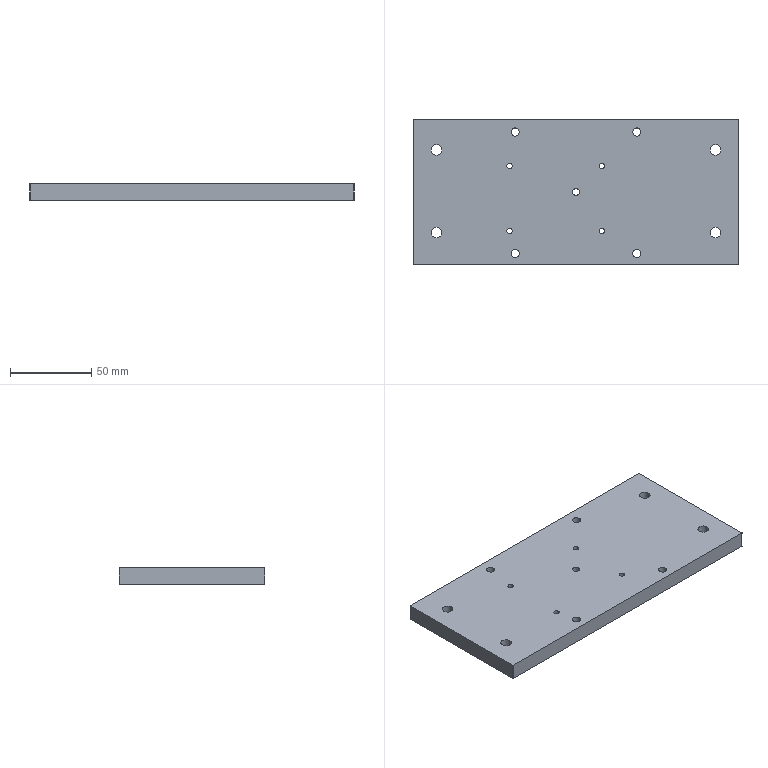CAM job | Mastercam | mm | 8 operations | part box 200 x 90 x 10
1. Facing | 20 - 63 平铣刀
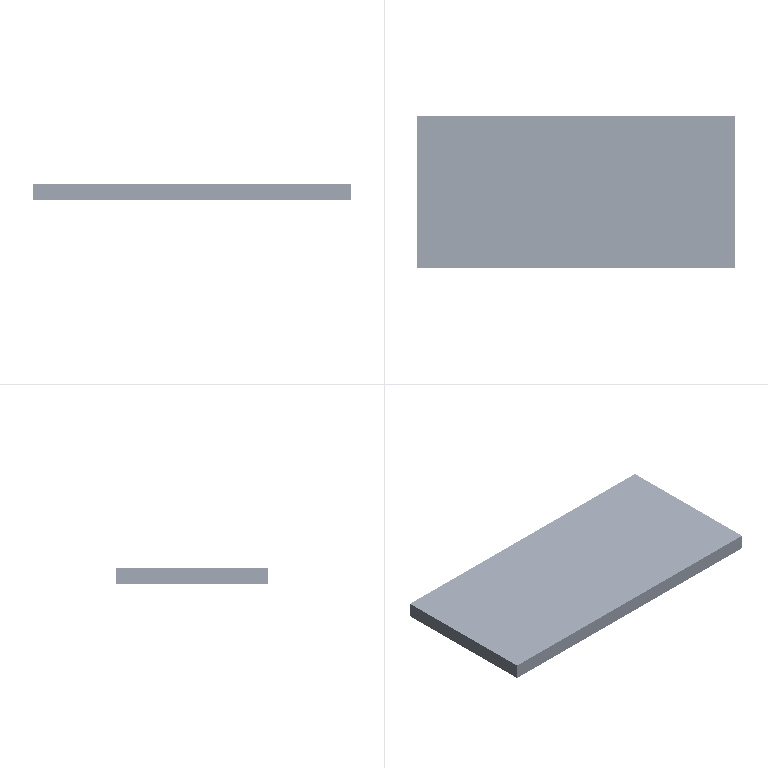2. Contour (Ramp) | 12 - 12 平铣刀
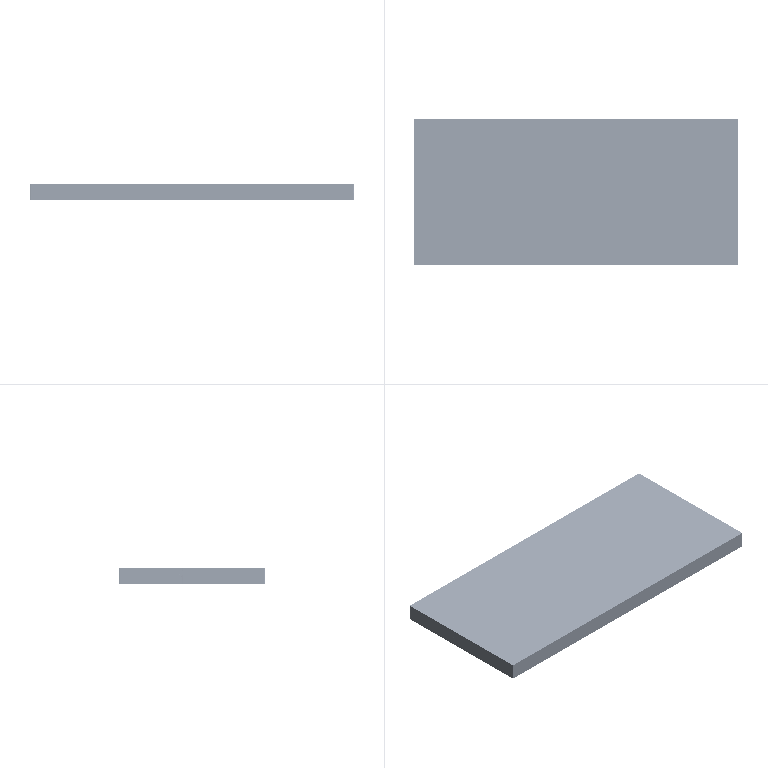3. Contour (2D) | 12 - 12 平铣刀
4. Drill/Counterbore | 7 - 4 倒角刀
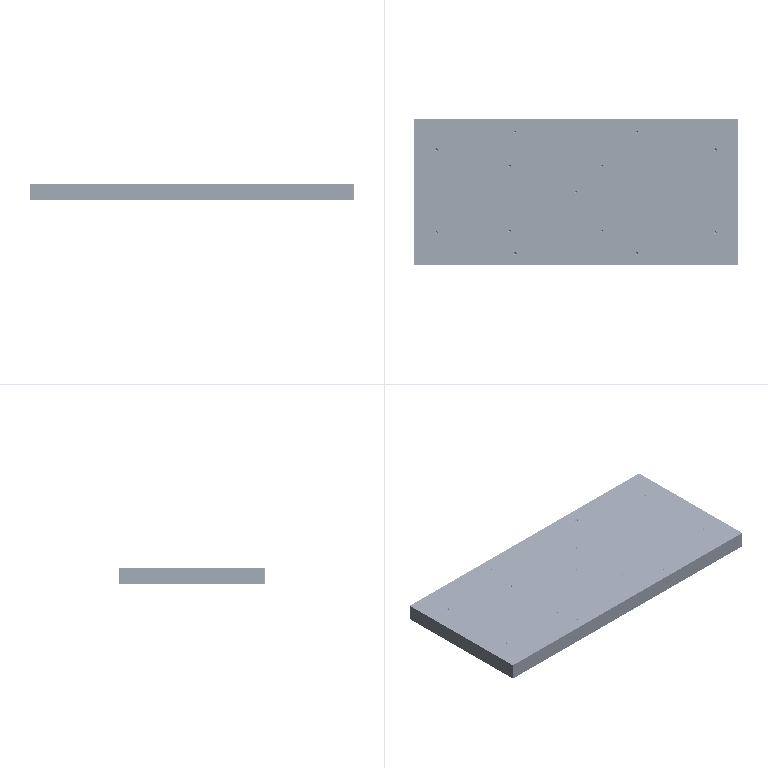5. Contour (2D chamfer) | 7 - 4 倒角刀
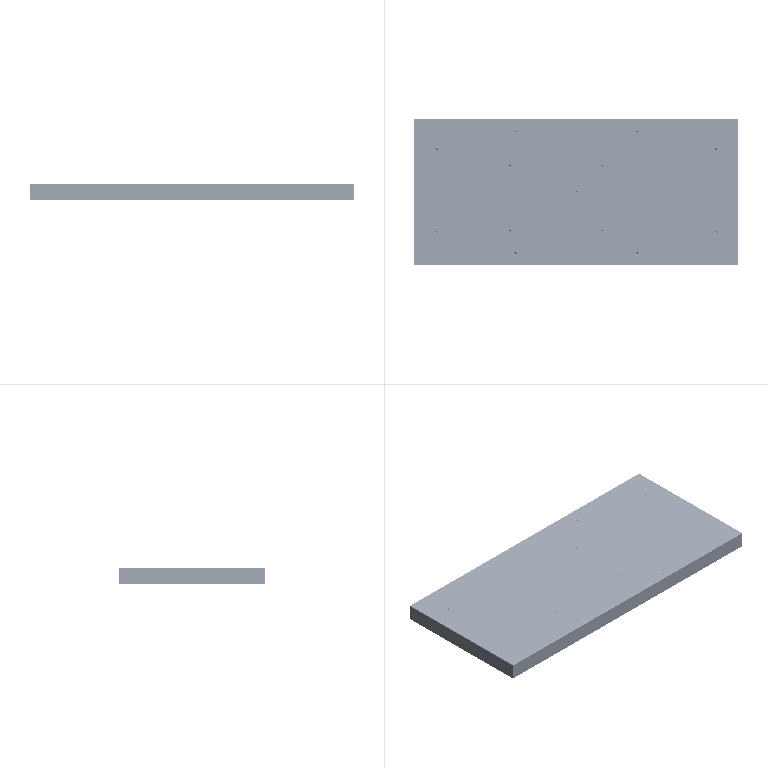6. Facing | 20 - 63 平铣刀
7. Contour (2D chamfer) | 7 - 4 倒角刀
8. Drill/Counterbore | 7 - 4 倒角刀